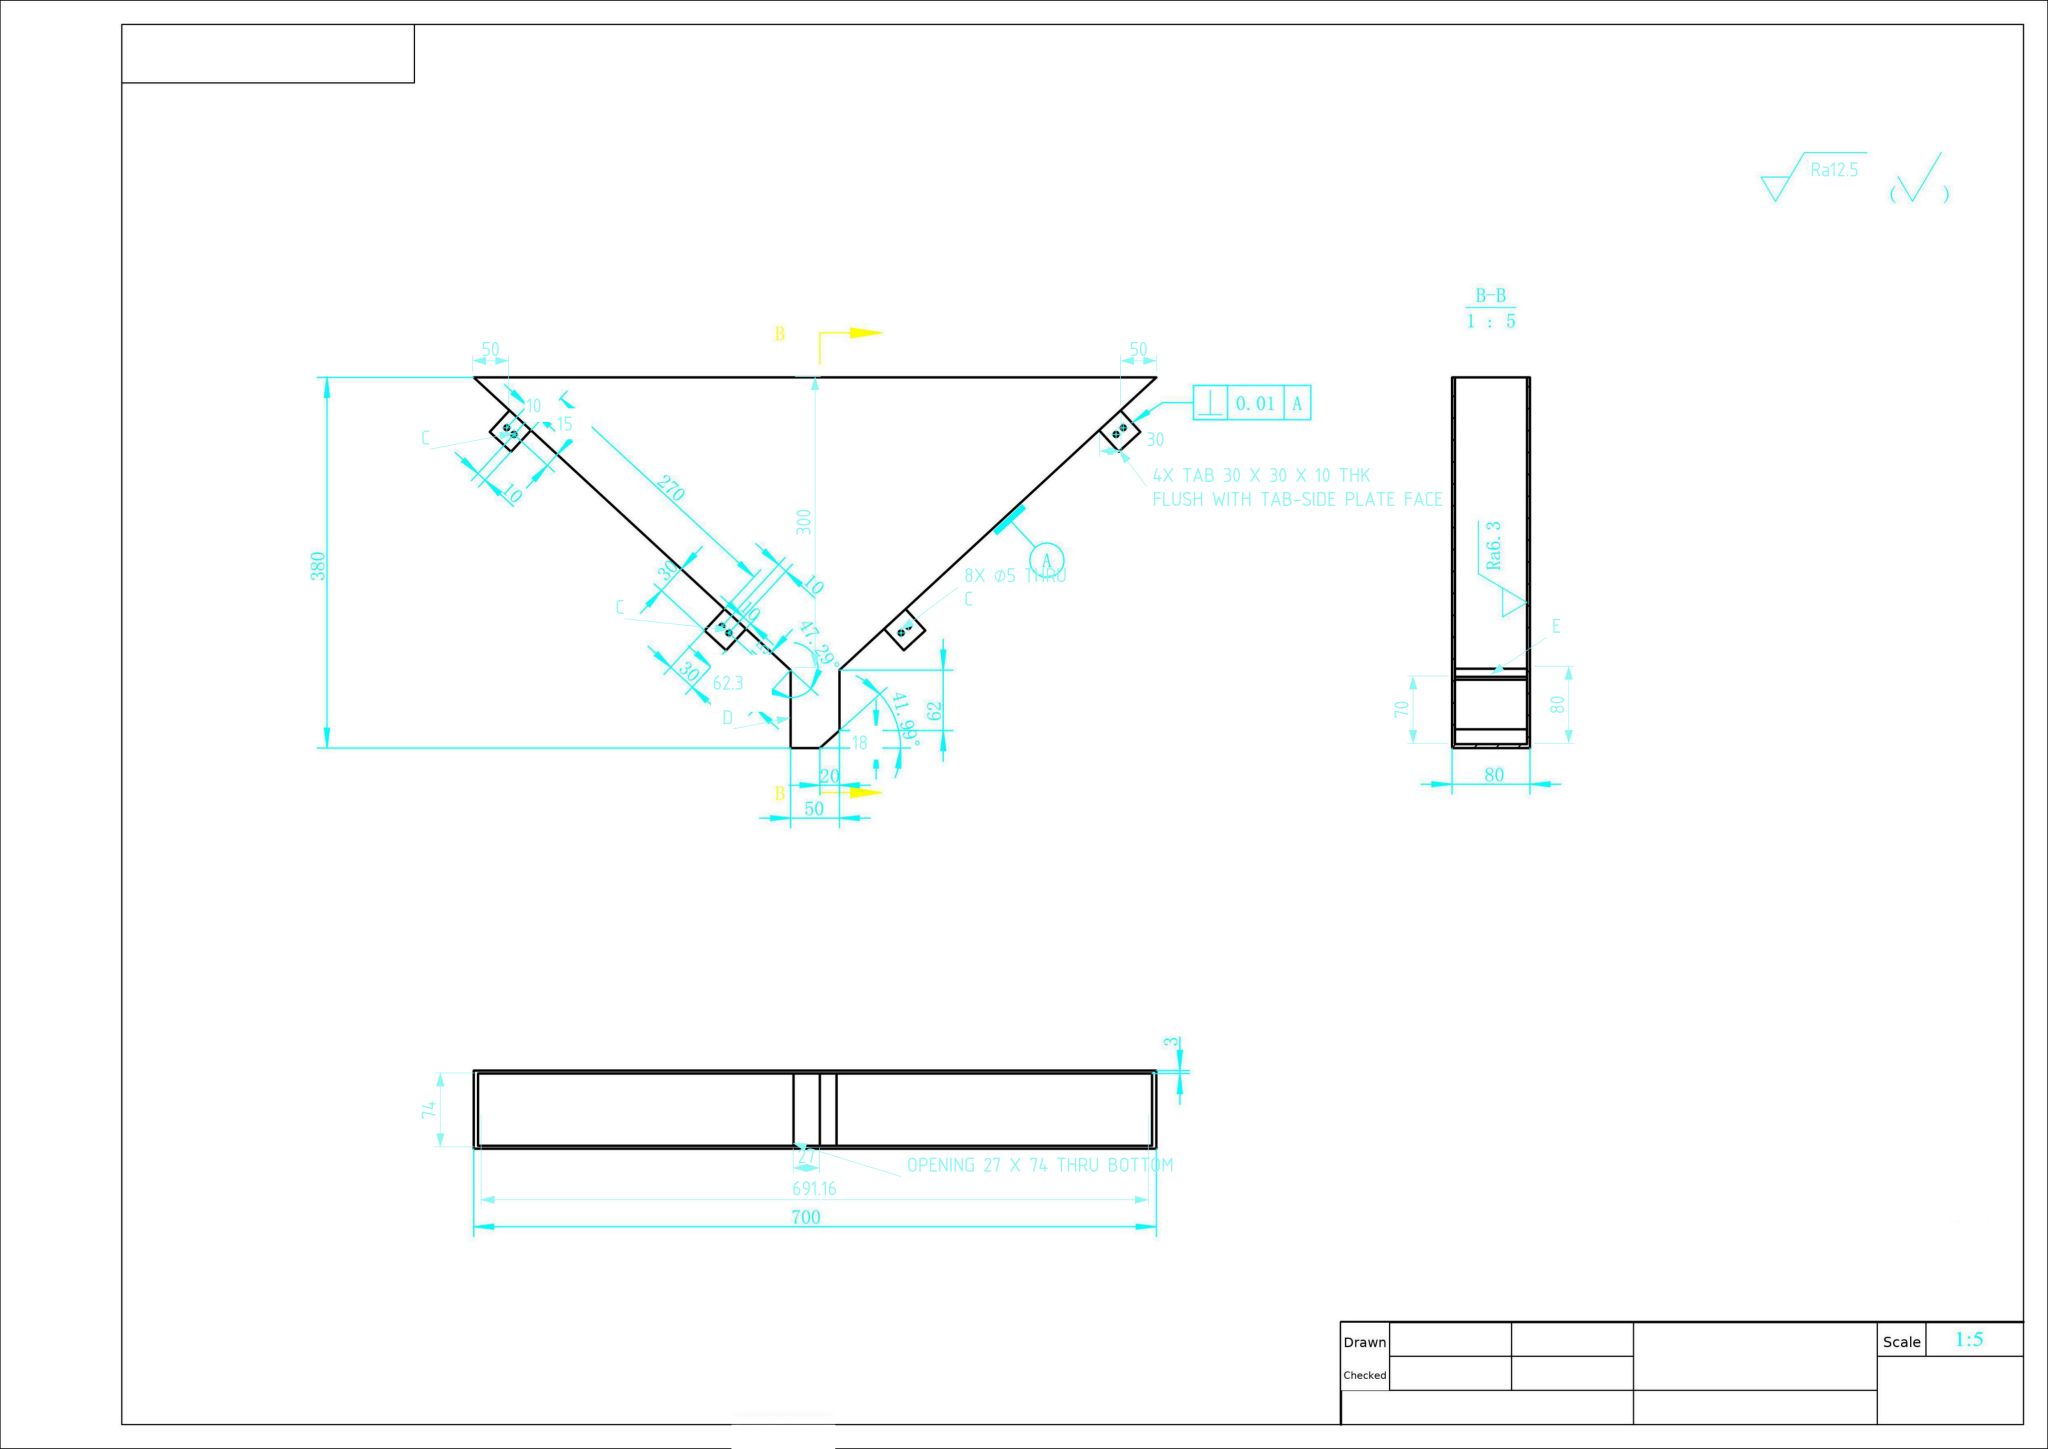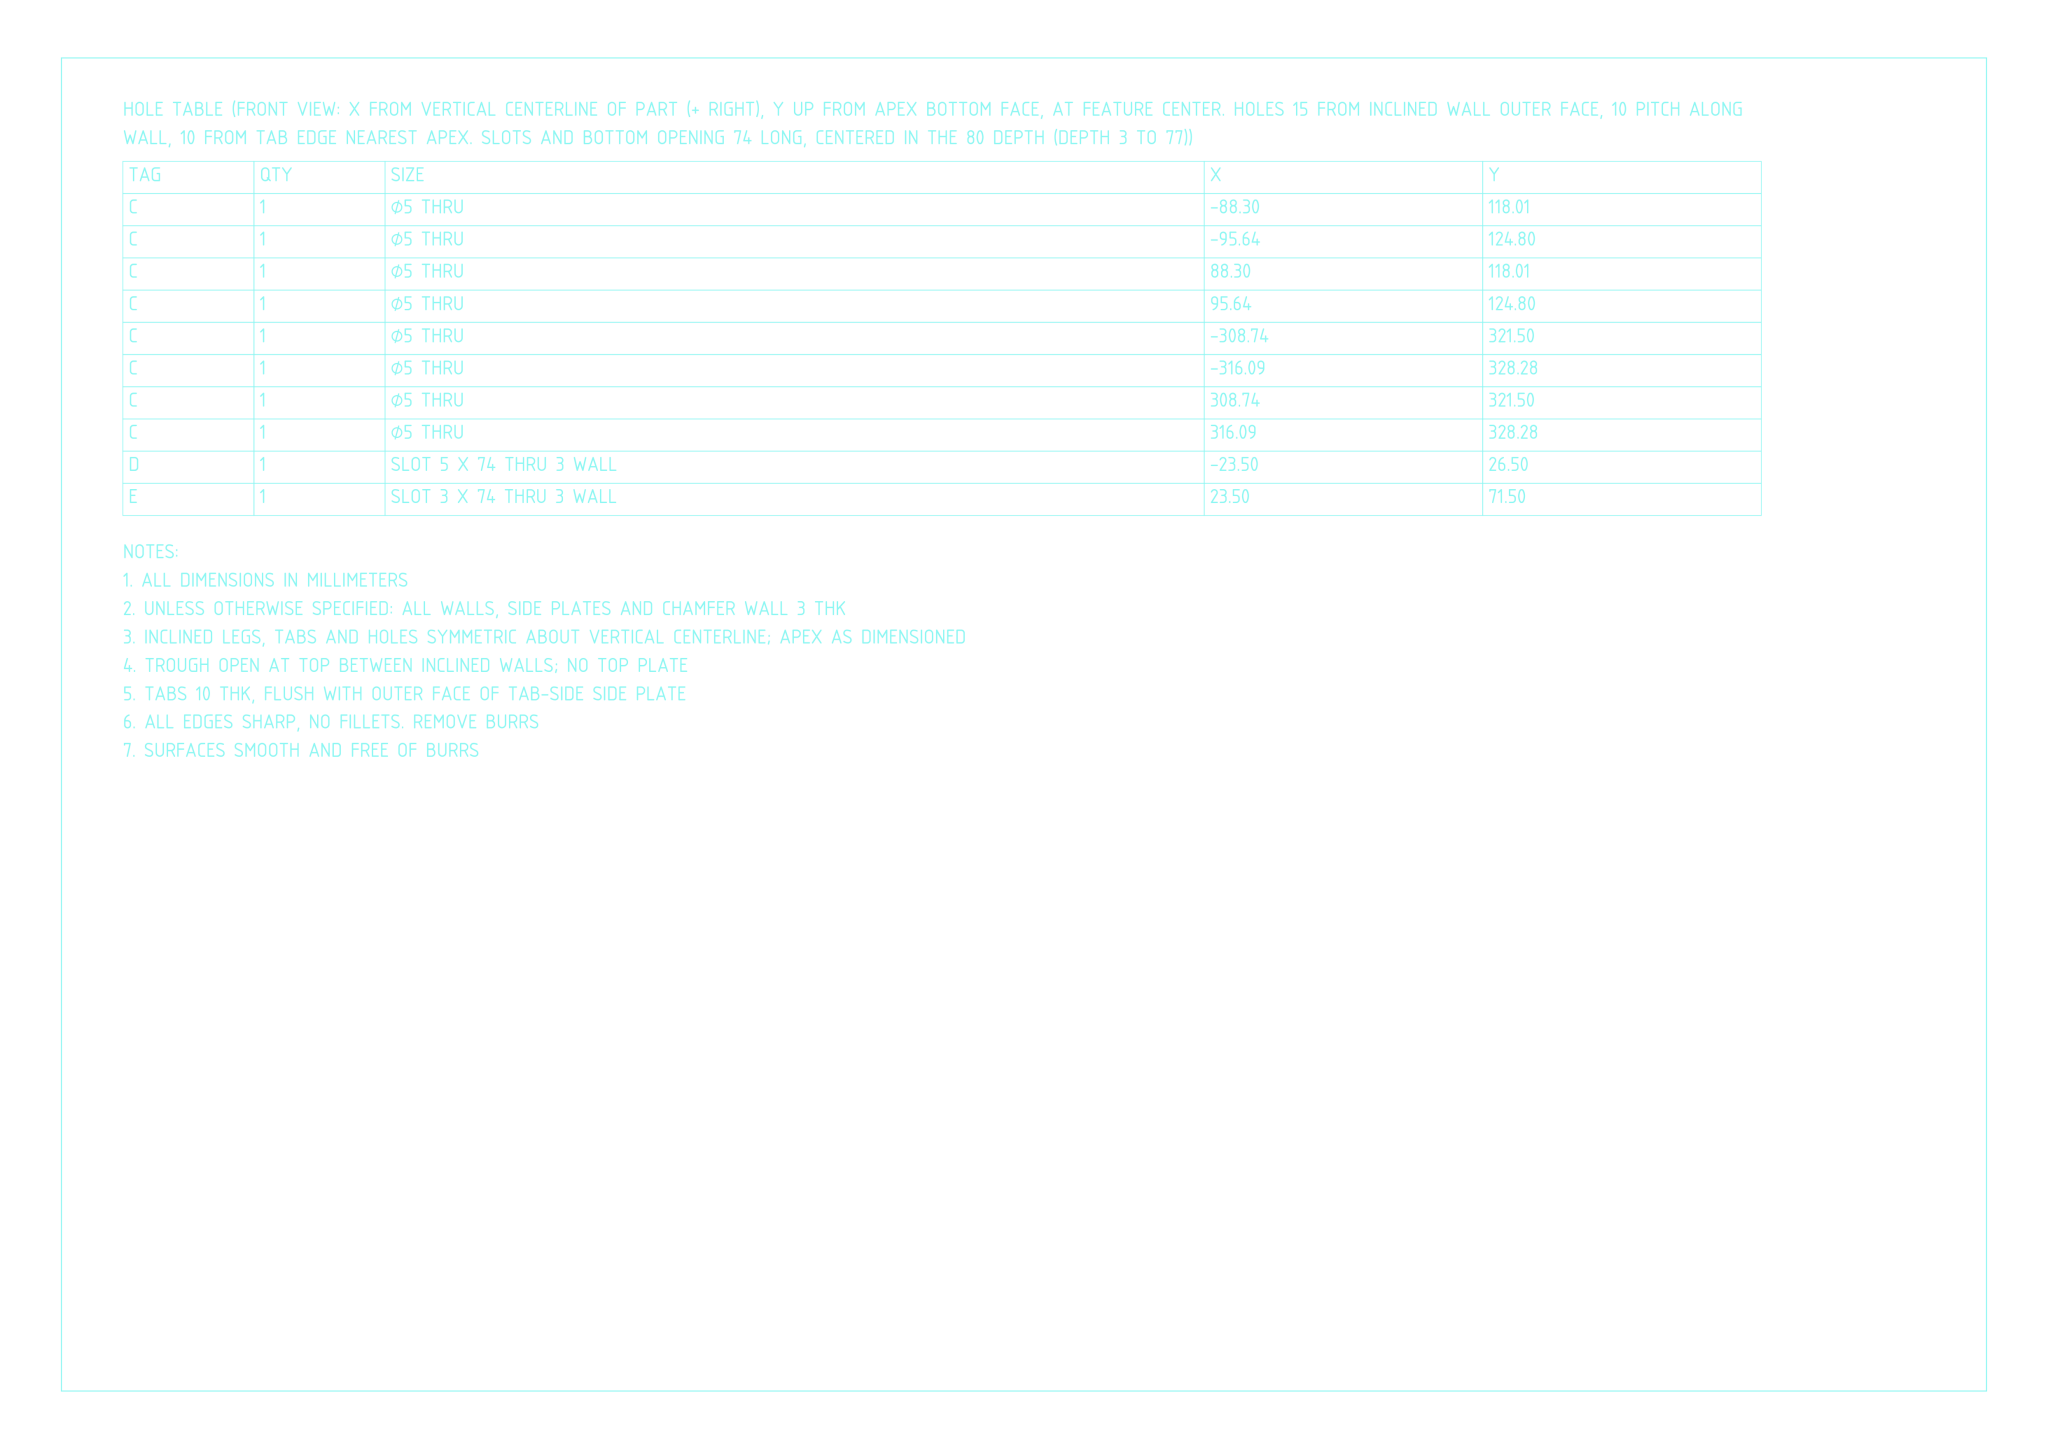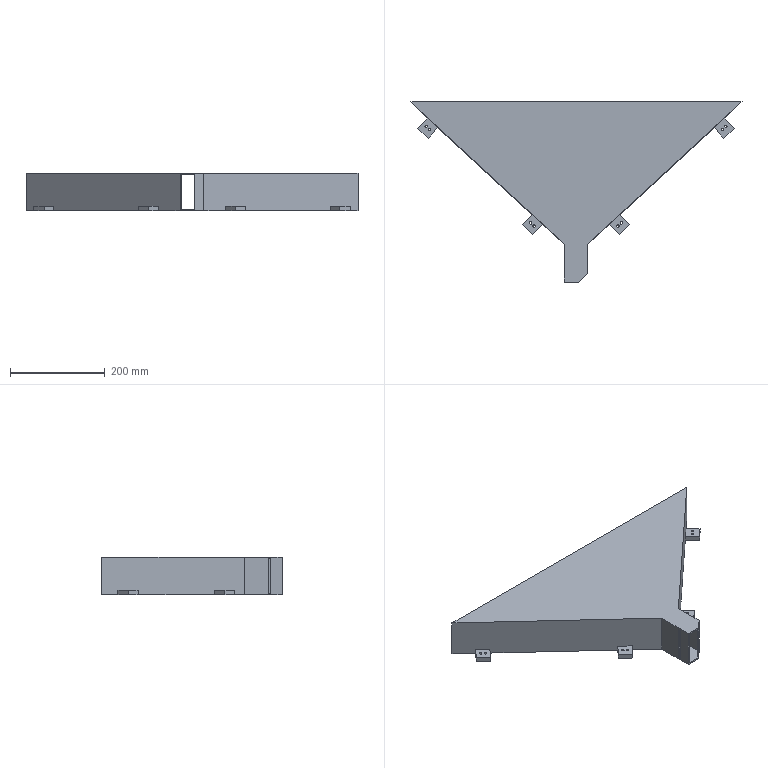Part | NX | mm | 1 solid | 55 faces | box 700 x 380 x 80 mm | volume 963715 mm3 | plane 39 | cylinder 16 | commonest cylinder face diameters 5 x16